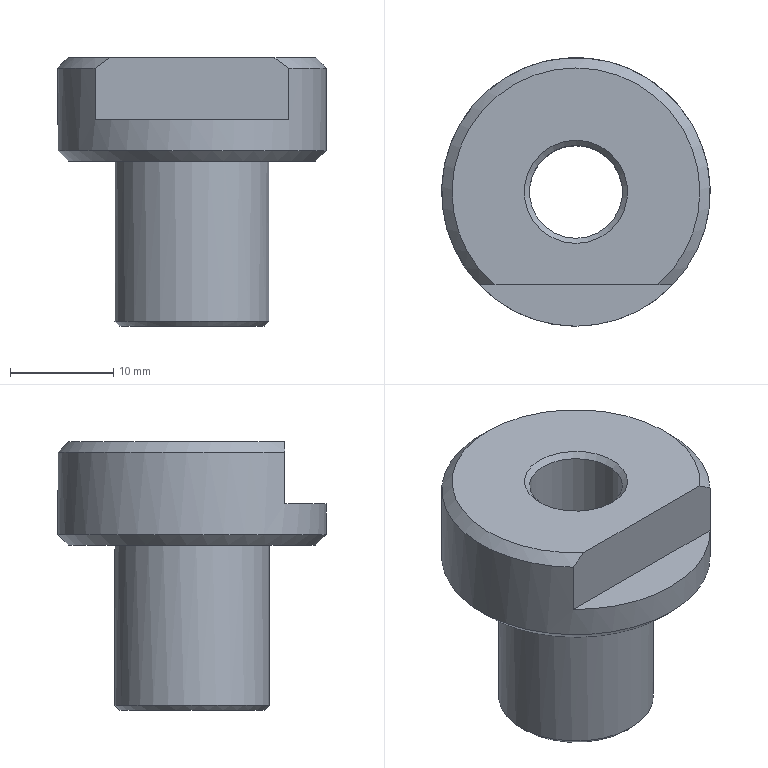Component | NX | DRILL_BUSHING | 1 solid | 13 faces | box 26 x 26 x 26 mm | volume 6089 mm3 | plane 5 | cone 5 | cylinder 3 | commonest cylinder face diameters 15 x1 26 x1 9 x1
STEP:
#1=CARTESIAN_POINT('',(0.,0.,0.));
#2=DIRECTION('',(0.,0.,1.));
#3=DIRECTION('',(1.,0.,0.));
#4=AXIS2_PLACEMENT_3D('',#1,#2,#3);
#5=CARTESIAN_POINT('',(376.101,-21.5,94.));
#6=VERTEX_POINT('',#5);
#7=CARTESIAN_POINT('',(376.101,-26.5,94.));
#8=DIRECTION('',(0.,0.,1.));
#9=DIRECTION('',(0.,1.,0.));
#10=AXIS2_PLACEMENT_3D('',#7,#8,#9);
#11=CIRCLE('',#10,5.);
#12=CARTESIAN_POINT('',(376.101,-26.5,94.));
#13=DIRECTION('',(0.,0.,-1.));
#14=DIRECTION('',(0.,1.,0.));
#15=AXIS2_PLACEMENT_3D('',#12,#13,#14);
#16=PLANE('',#15);
#17=CARTESIAN_POINT('',(5.,0.));
#18=CARTESIAN_POINT('',(5.,-8.66));
#19=CARTESIAN_POINT('',(-2.5,-4.33));
#20=CARTESIAN_POINT('',(-10.,-0.));
#21=CARTESIAN_POINT('',(-2.5,4.33));
#22=CARTESIAN_POINT('',(5.,8.66));
#23=CARTESIAN_POINT('',(5.,0.));
#24=(BOUNDED_CURVE()B_SPLINE_CURVE(2,(#17,#18,#19,#20,#21,#22,#23),.UNSPECIFIED.,.T.,.F.)B_SPLINE_CURVE_WITH_KNOTS((1,2,2,2,2,1),(-2.094,0.,2.094,4.189,6.283,8.378),.UNSPECIFIED.)CURVE()GEOMETRIC_REPRESENTATION_ITEM()RATIONAL_B_SPLINE_CURVE((1.,0.5,1.,0.5,1.,0.5,1.))REPRESENTATION_ITEM(''));
#25=(GEOMETRIC_REPRESENTATION_CONTEXT(2)PARAMETRIC_REPRESENTATION_CONTEXT()REPRESENTATION_CONTEXT('',''));
#26=DEFINITIONAL_REPRESENTATION('',(#24),#25);
#27=PCURVE('',#16,#26);
#28=CARTESIAN_POINT('',(376.101,-26.5,94.5));
#29=DIRECTION('',(0.,0.,-1.));
#30=DIRECTION('',(0.,1.,0.));
#31=AXIS2_PLACEMENT_3D('',#28,#29,#30);
#32=CONICAL_SURFACE('',#31,4.5,0.7854);
#33=CARTESIAN_POINT('',(6.283,0.5));
#34=DIRECTION('',(-1.,0.));
#35=VECTOR('',#34,1.);
#36=LINE('',#33,#35);
#37=(GEOMETRIC_REPRESENTATION_CONTEXT(2)PARAMETRIC_REPRESENTATION_CONTEXT()REPRESENTATION_CONTEXT('',''));
#38=DEFINITIONAL_REPRESENTATION('',(#36),#37);
#39=PCURVE('',#32,#38);
#40=SURFACE_CURVE('',#11,(#27,#39),.PCURVE_S1.);
#41=EDGE_CURVE('',#6,#6,#40,.T.);
#42=ORIENTED_EDGE('',*,*,#41,.T.);
#43=EDGE_LOOP('',(#42));
#44=FACE_BOUND('',#43,.T.);
#45=CARTESIAN_POINT('',(376.101,-19.5,94.));
#46=VERTEX_POINT('',#45);
#47=CARTESIAN_POINT('',(376.101,-26.5,94.));
#48=DIRECTION('',(0.,0.,-1.));
#49=DIRECTION('',(0.,1.,0.));
#50=AXIS2_PLACEMENT_3D('',#47,#48,#49);
#51=CIRCLE('',#50,7.);
#52=CARTESIAN_POINT('',(0.,0.));
#53=DIRECTION('',(1.,0.));
#54=AXIS2_PLACEMENT_2D('',#52,#53);
#55=CIRCLE('',#54,7.);
#56=(GEOMETRIC_REPRESENTATION_CONTEXT(2)PARAMETRIC_REPRESENTATION_CONTEXT()REPRESENTATION_CONTEXT('',''));
#57=DEFINITIONAL_REPRESENTATION('',(#55),#56);
#58=PCURVE('',#16,#57);
#59=CARTESIAN_POINT('',(376.101,-26.5,94.5));
#60=DIRECTION('',(0.,0.,1.));
#61=DIRECTION('',(0.,-1.,0.));
#62=AXIS2_PLACEMENT_3D('',#59,#60,#61);
#63=CONICAL_SURFACE('',#62,7.5,0.7854);
#64=CARTESIAN_POINT('',(9.425,-0.5));
#65=DIRECTION('',(-1.,0.));
#66=VECTOR('',#65,1.);
#67=LINE('',#64,#66);
#68=(GEOMETRIC_REPRESENTATION_CONTEXT(2)PARAMETRIC_REPRESENTATION_CONTEXT()REPRESENTATION_CONTEXT('',''));
#69=DEFINITIONAL_REPRESENTATION('',(#67),#68);
#70=PCURVE('',#63,#69);
#71=SURFACE_CURVE('',#51,(#58,#70),.PCURVE_S1.);
#72=EDGE_CURVE('',#46,#46,#71,.T.);
#73=ORIENTED_EDGE('',*,*,#72,.T.);
#74=EDGE_LOOP('',(#73));
#75=FACE_BOUND('',#74,.T.);
#76=ADVANCED_FACE('',(#44,#75),#16,.T.);
#77=CARTESIAN_POINT('',(376.101,-19.,94.5));
#78=VERTEX_POINT('',#77);
#79=CARTESIAN_POINT('',(376.101,-34.,94.5));
#80=VERTEX_POINT('',#79);
#81=CARTESIAN_POINT('',(376.101,-26.5,94.5));
#82=DIRECTION('',(0.,0.,1.));
#83=DIRECTION('',(0.,1.,0.));
#84=AXIS2_PLACEMENT_3D('',#81,#82,#83);
#85=CIRCLE('',#84,7.5);
#86=CARTESIAN_POINT('',(376.101,-26.5,94.));
#87=DIRECTION('',(0.,0.,1.));
#88=DIRECTION('',(0.,-1.,0.));
#89=AXIS2_PLACEMENT_3D('',#86,#87,#88);
#90=CYLINDRICAL_SURFACE('',#89,7.5);
#91=CARTESIAN_POINT('',(3.142,0.5));
#92=DIRECTION('',(1.,0.));
#93=VECTOR('',#92,1.);
#94=LINE('',#91,#93);
#95=(GEOMETRIC_REPRESENTATION_CONTEXT(2)PARAMETRIC_REPRESENTATION_CONTEXT()REPRESENTATION_CONTEXT('',''));
#96=DEFINITIONAL_REPRESENTATION('',(#94),#95);
#97=PCURVE('',#90,#96);
#98=CARTESIAN_POINT('',(3.142,0.));
#99=DIRECTION('',(1.,0.));
#100=VECTOR('',#99,1.);
#101=LINE('',#98,#100);
#102=(GEOMETRIC_REPRESENTATION_CONTEXT(2)PARAMETRIC_REPRESENTATION_CONTEXT()REPRESENTATION_CONTEXT('',''));
#103=DEFINITIONAL_REPRESENTATION('',(#101),#102);
#104=PCURVE('',#63,#103);
#105=SURFACE_CURVE('',#85,(#97,#104),.PCURVE_S1.);
#106=EDGE_CURVE('',#78,#80,#105,.T.);
#107=ORIENTED_EDGE('',*,*,#106,.T.);
#108=CARTESIAN_POINT('',(376.101,-34.,110.));
#109=VERTEX_POINT('',#108);
#110=CARTESIAN_POINT('',(376.101,-34.,94.5));
#111=CARTESIAN_POINT('',(376.101,-34.,110.));
#112=B_SPLINE_CURVE_WITH_KNOTS('',1,(#110,#111),.UNSPECIFIED.,.F.,.F.,(2,2),(0.5,16.),.PIECEWISE_BEZIER_KNOTS.);
#113=CARTESIAN_POINT('',(6.283,0.));
#114=DIRECTION('',(0.,1.));
#115=VECTOR('',#114,1.);
#116=LINE('',#113,#115);
#117=(GEOMETRIC_REPRESENTATION_CONTEXT(2)PARAMETRIC_REPRESENTATION_CONTEXT()REPRESENTATION_CONTEXT('',''));
#118=DEFINITIONAL_REPRESENTATION('',(#116),#117);
#119=PCURVE('',#90,#118);
#120=CARTESIAN_POINT('',(0.,0.));
#121=DIRECTION('',(0.,1.));
#122=VECTOR('',#121,1.);
#123=LINE('',#120,#122);
#124=(GEOMETRIC_REPRESENTATION_CONTEXT(2)PARAMETRIC_REPRESENTATION_CONTEXT()REPRESENTATION_CONTEXT('',''));
#125=DEFINITIONAL_REPRESENTATION('',(#123),#124);
#126=PCURVE('',#90,#125);
#127=SEAM_CURVE('',#112,(#119,#126),.PCURVE_S1.);
#128=EDGE_CURVE('',#80,#109,#127,.T.);
#129=ORIENTED_EDGE('',*,*,#128,.T.);
#130=CARTESIAN_POINT('',(376.101,-26.5,110.));
#131=DIRECTION('',(0.,0.,-1.));
#132=DIRECTION('',(0.,-1.,0.));
#133=AXIS2_PLACEMENT_3D('',#130,#131,#132);
#134=CIRCLE('',#133,7.5);
#135=CARTESIAN_POINT('',(6.283,16.));
#136=DIRECTION('',(-1.,0.));
#137=VECTOR('',#136,1.);
#138=LINE('',#135,#137);
#139=(GEOMETRIC_REPRESENTATION_CONTEXT(2)PARAMETRIC_REPRESENTATION_CONTEXT()REPRESENTATION_CONTEXT('',''));
#140=DEFINITIONAL_REPRESENTATION('',(#138),#139);
#141=PCURVE('',#90,#140);
#142=CARTESIAN_POINT('',(376.101,-26.5,110.));
#143=DIRECTION('',(0.,0.,-1.));
#144=DIRECTION('',(0.,1.,0.));
#145=AXIS2_PLACEMENT_3D('',#142,#143,#144);
#146=PLANE('',#145);
#147=CARTESIAN_POINT('',(0.,0.));
#148=DIRECTION('',(-1.,0.));
#149=AXIS2_PLACEMENT_2D('',#147,#148);
#150=CIRCLE('',#149,7.5);
#151=(GEOMETRIC_REPRESENTATION_CONTEXT(2)PARAMETRIC_REPRESENTATION_CONTEXT()REPRESENTATION_CONTEXT('',''));
#152=DEFINITIONAL_REPRESENTATION('',(#150),#151);
#153=PCURVE('',#146,#152);
#154=SURFACE_CURVE('',#134,(#141,#153),.PCURVE_S1.);
#155=EDGE_CURVE('',#109,#109,#154,.T.);
#156=ORIENTED_EDGE('',*,*,#155,.T.);
#157=ORIENTED_EDGE('',*,*,#128,.F.);
#158=CARTESIAN_POINT('',(376.101,-26.5,94.5));
#159=DIRECTION('',(0.,0.,1.));
#160=DIRECTION('',(0.,1.,0.));
#161=AXIS2_PLACEMENT_3D('',#158,#159,#160);
#162=CIRCLE('',#161,7.5);
#163=CARTESIAN_POINT('',(-3.142,0.5));
#164=DIRECTION('',(1.,0.));
#165=VECTOR('',#164,1.);
#166=LINE('',#163,#165);
#167=(GEOMETRIC_REPRESENTATION_CONTEXT(2)PARAMETRIC_REPRESENTATION_CONTEXT()REPRESENTATION_CONTEXT('',''));
#168=DEFINITIONAL_REPRESENTATION('',(#166),#167);
#169=PCURVE('',#90,#168);
#170=CARTESIAN_POINT('',(3.142,0.));
#171=DIRECTION('',(1.,0.));
#172=VECTOR('',#171,1.);
#173=LINE('',#170,#172);
#174=(GEOMETRIC_REPRESENTATION_CONTEXT(2)PARAMETRIC_REPRESENTATION_CONTEXT()REPRESENTATION_CONTEXT('',''));
#175=DEFINITIONAL_REPRESENTATION('',(#173),#174);
#176=PCURVE('',#63,#175);
#177=SURFACE_CURVE('',#162,(#169,#176),.PCURVE_S1.);
#178=EDGE_CURVE('',#80,#78,#177,.T.);
#179=ORIENTED_EDGE('',*,*,#178,.T.);
#180=EDGE_LOOP('',(#107,#129,#156,#157,#179));
#181=FACE_BOUND('',#180,.T.);
#182=ADVANCED_FACE('',(#181),#90,.T.);
#183=CARTESIAN_POINT('',(376.101,-31.5,120.));
#184=VERTEX_POINT('',#183);
#185=CARTESIAN_POINT('',(376.101,-26.5,120.));
#186=DIRECTION('',(0.,0.,-1.));
#187=DIRECTION('',(0.,-1.,0.));
#188=AXIS2_PLACEMENT_3D('',#185,#186,#187);
#189=CIRCLE('',#188,5.);
#190=CARTESIAN_POINT('',(376.101,-26.5,120.));
#191=DIRECTION('',(0.,0.,1.));
#192=DIRECTION('',(0.,-1.,0.));
#193=AXIS2_PLACEMENT_3D('',#190,#191,#192);
#194=PLANE('',#193);
#195=CARTESIAN_POINT('',(5.,0.));
#196=CARTESIAN_POINT('',(5.,-8.66));
#197=CARTESIAN_POINT('',(-2.5,-4.33));
#198=CARTESIAN_POINT('',(-10.,-0.));
#199=CARTESIAN_POINT('',(-2.5,4.33));
#200=CARTESIAN_POINT('',(5.,8.66));
#201=CARTESIAN_POINT('',(5.,0.));
#202=(BOUNDED_CURVE()B_SPLINE_CURVE(2,(#195,#196,#197,#198,#199,#200,#201),.UNSPECIFIED.,.T.,.F.)B_SPLINE_CURVE_WITH_KNOTS((1,2,2,2,2,1),(-2.094,0.,2.094,4.189,6.283,8.378),.UNSPECIFIED.)CURVE()GEOMETRIC_REPRESENTATION_ITEM()RATIONAL_B_SPLINE_CURVE((1.,0.5,1.,0.5,1.,0.5,1.))REPRESENTATION_ITEM(''));
#203=(GEOMETRIC_REPRESENTATION_CONTEXT(2)PARAMETRIC_REPRESENTATION_CONTEXT()REPRESENTATION_CONTEXT('',''));
#204=DEFINITIONAL_REPRESENTATION('',(#202),#203);
#205=PCURVE('',#194,#204);
#206=CARTESIAN_POINT('',(376.101,-26.5,120.));
#207=DIRECTION('',(0.,0.,1.));
#208=DIRECTION('',(0.,-1.,0.));
#209=AXIS2_PLACEMENT_3D('',#206,#207,#208);
#210=CONICAL_SURFACE('',#209,5.,0.7854);
#211=CARTESIAN_POINT('',(6.283,0.));
#212=DIRECTION('',(-1.,0.));
#213=VECTOR('',#212,1.);
#214=LINE('',#211,#213);
#215=(GEOMETRIC_REPRESENTATION_CONTEXT(2)PARAMETRIC_REPRESENTATION_CONTEXT()REPRESENTATION_CONTEXT('',''));
#216=DEFINITIONAL_REPRESENTATION('',(#214),#215);
#217=PCURVE('',#210,#216);
#218=SURFACE_CURVE('',#189,(#205,#217),.PCURVE_S1.);
#219=EDGE_CURVE('',#184,#184,#218,.T.);
#220=ORIENTED_EDGE('',*,*,#219,.T.);
#221=EDGE_LOOP('',(#220));
#222=FACE_BOUND('',#221,.T.);
#223=CARTESIAN_POINT('',(384.038,-35.5,120.));
#224=VERTEX_POINT('',#223);
#225=CARTESIAN_POINT('',(368.164,-35.5,120.));
#226=VERTEX_POINT('',#225);
#227=CARTESIAN_POINT('',(399.244,-35.5,120.));
#228=DIRECTION('',(-1.,0.,0.));
#229=VECTOR('',#228,1.);
#230=LINE('',#227,#229);
#231=CARTESIAN_POINT('',(9.,23.143));
#232=DIRECTION('',(0.,-1.));
#233=VECTOR('',#232,1.);
#234=LINE('',#231,#233);
#235=(GEOMETRIC_REPRESENTATION_CONTEXT(2)PARAMETRIC_REPRESENTATION_CONTEXT()REPRESENTATION_CONTEXT('',''));
#236=DEFINITIONAL_REPRESENTATION('',(#234),#235);
#237=PCURVE('',#194,#236);
#238=CARTESIAN_POINT('',(399.244,-35.5,114.));
#239=DIRECTION('',(0.,1.,0.));
#240=DIRECTION('',(0.,0.,1.));
#241=AXIS2_PLACEMENT_3D('',#238,#239,#240);
#242=PLANE('',#241);
#243=CARTESIAN_POINT('',(6.,0.));
#244=DIRECTION('',(0.,-1.));
#245=VECTOR('',#244,1.);
#246=LINE('',#243,#245);
#247=(GEOMETRIC_REPRESENTATION_CONTEXT(2)PARAMETRIC_REPRESENTATION_CONTEXT()REPRESENTATION_CONTEXT('',''));
#248=DEFINITIONAL_REPRESENTATION('',(#246),#247);
#249=PCURVE('',#242,#248);
#250=SURFACE_CURVE('',#230,(#237,#249),.PCURVE_S1.);
#251=EDGE_CURVE('',#224,#226,#250,.T.);
#252=ORIENTED_EDGE('',*,*,#251,.F.);
#253=CARTESIAN_POINT('',(376.101,-26.5,120.));
#254=DIRECTION('',(0.,0.,1.));
#255=DIRECTION('',(0.,-1.,0.));
#256=AXIS2_PLACEMENT_3D('',#253,#254,#255);
#257=CIRCLE('',#256,12.);
#258=CARTESIAN_POINT('',(0.,0.));
#259=DIRECTION('',(1.,0.));
#260=AXIS2_PLACEMENT_2D('',#258,#259);
#261=CIRCLE('',#260,12.);
#262=(GEOMETRIC_REPRESENTATION_CONTEXT(2)PARAMETRIC_REPRESENTATION_CONTEXT()REPRESENTATION_CONTEXT('',''));
#263=DEFINITIONAL_REPRESENTATION('',(#261),#262);
#264=PCURVE('',#194,#263);
#265=CARTESIAN_POINT('',(376.101,-26.5,119.));
#266=DIRECTION('',(0.,0.,-1.));
#267=DIRECTION('',(0.,1.,0.));
#268=AXIS2_PLACEMENT_3D('',#265,#266,#267);
#269=CONICAL_SURFACE('',#268,13.,0.7854);
#270=CARTESIAN_POINT('',(9.425,-1.));
#271=DIRECTION('',(-1.,0.));
#272=VECTOR('',#271,1.);
#273=LINE('',#270,#272);
#274=(GEOMETRIC_REPRESENTATION_CONTEXT(2)PARAMETRIC_REPRESENTATION_CONTEXT()REPRESENTATION_CONTEXT('',''));
#275=DEFINITIONAL_REPRESENTATION('',(#273),#274);
#276=PCURVE('',#269,#275);
#277=SURFACE_CURVE('',#257,(#264,#276),.PCURVE_S1.);
#278=EDGE_CURVE('',#224,#226,#277,.T.);
#279=ORIENTED_EDGE('',*,*,#278,.T.);
#280=EDGE_LOOP('',(#252,#279));
#281=FACE_BOUND('',#280,.T.);
#282=ADVANCED_FACE('',(#222,#281),#194,.T.);
#283=CARTESIAN_POINT('',(376.101,-14.5,110.));
#284=VERTEX_POINT('',#283);
#285=CARTESIAN_POINT('',(376.101,-26.5,110.));
#286=DIRECTION('',(0.,0.,-1.));
#287=DIRECTION('',(0.,1.,0.));
#288=AXIS2_PLACEMENT_3D('',#285,#286,#287);
#289=CIRCLE('',#288,12.);
#290=CARTESIAN_POINT('',(0.,0.));
#291=DIRECTION('',(1.,0.));
#292=AXIS2_PLACEMENT_2D('',#290,#291);
#293=CIRCLE('',#292,12.);
#294=(GEOMETRIC_REPRESENTATION_CONTEXT(2)PARAMETRIC_REPRESENTATION_CONTEXT()REPRESENTATION_CONTEXT('',''));
#295=DEFINITIONAL_REPRESENTATION('',(#293),#294);
#296=PCURVE('',#146,#295);
#297=CARTESIAN_POINT('',(376.101,-26.5,111.));
#298=DIRECTION('',(0.,0.,1.));
#299=DIRECTION('',(0.,-1.,0.));
#300=AXIS2_PLACEMENT_3D('',#297,#298,#299);
#301=CONICAL_SURFACE('',#300,13.,0.7854);
#302=CARTESIAN_POINT('',(9.425,-1.));
#303=DIRECTION('',(-1.,0.));
#304=VECTOR('',#303,1.);
#305=LINE('',#302,#304);
#306=(GEOMETRIC_REPRESENTATION_CONTEXT(2)PARAMETRIC_REPRESENTATION_CONTEXT()REPRESENTATION_CONTEXT('',''));
#307=DEFINITIONAL_REPRESENTATION('',(#305),#306);
#308=PCURVE('',#301,#307);
#309=SURFACE_CURVE('',#289,(#296,#308),.PCURVE_S1.);
#310=EDGE_CURVE('',#284,#284,#309,.T.);
#311=ORIENTED_EDGE('',*,*,#310,.T.);
#312=EDGE_LOOP('',(#311));
#313=FACE_BOUND('',#312,.T.);
#314=ORIENTED_EDGE('',*,*,#155,.F.);
#315=EDGE_LOOP('',(#314));
#316=FACE_BOUND('',#315,.T.);
#317=ADVANCED_FACE('',(#313,#316),#146,.T.);
#318=CARTESIAN_POINT('',(376.101,-13.5,111.));
#319=VERTEX_POINT('',#318);
#320=CARTESIAN_POINT('',(385.482,-35.5,111.));
#321=VERTEX_POINT('',#320);
#322=CARTESIAN_POINT('',(376.101,-26.5,111.));
#323=DIRECTION('',(0.,0.,1.));
#324=DIRECTION('',(0.,1.,0.));
#325=AXIS2_PLACEMENT_3D('',#322,#323,#324);
#326=CIRCLE('',#325,13.);
#327=CARTESIAN_POINT('',(376.101,-26.5,110.));
#328=DIRECTION('',(0.,0.,1.));
#329=DIRECTION('',(0.,-1.,0.));
#330=AXIS2_PLACEMENT_3D('',#327,#328,#329);
#331=CYLINDRICAL_SURFACE('',#330,13.);
#332=CARTESIAN_POINT('',(3.142,1.));
#333=DIRECTION('',(1.,0.));
#334=VECTOR('',#333,1.);
#335=LINE('',#332,#334);
#336=(GEOMETRIC_REPRESENTATION_CONTEXT(2)PARAMETRIC_REPRESENTATION_CONTEXT()REPRESENTATION_CONTEXT('',''));
#337=DEFINITIONAL_REPRESENTATION('',(#335),#336);
#338=PCURVE('',#331,#337);
#339=CARTESIAN_POINT('',(3.142,0.));
#340=DIRECTION('',(1.,-0.));
#341=VECTOR('',#340,1.);
#342=LINE('',#339,#341);
#343=(GEOMETRIC_REPRESENTATION_CONTEXT(2)PARAMETRIC_REPRESENTATION_CONTEXT()REPRESENTATION_CONTEXT('',''));
#344=DEFINITIONAL_REPRESENTATION('',(#342),#343);
#345=PCURVE('',#301,#344);
#346=SURFACE_CURVE('',#326,(#338,#345),.PCURVE_S1.);
#347=EDGE_CURVE('',#319,#321,#346,.T.);
#348=ORIENTED_EDGE('',*,*,#347,.T.);
#349=CARTESIAN_POINT('',(385.482,-35.5,114.));
#350=VERTEX_POINT('',#349);
#351=CARTESIAN_POINT('',(385.482,-35.5,111.));
#352=CARTESIAN_POINT('',(385.482,-35.5,114.));
#353=B_SPLINE_CURVE_WITH_KNOTS('',1,(#351,#352),.UNSPECIFIED.,.F.,.F.,(2,2),(1.,4.),.PIECEWISE_BEZIER_KNOTS.);
#354=CARTESIAN_POINT('',(7.089,0.));
#355=DIRECTION('',(0.,1.));
#356=VECTOR('',#355,1.);
#357=LINE('',#354,#356);
#358=(GEOMETRIC_REPRESENTATION_CONTEXT(2)PARAMETRIC_REPRESENTATION_CONTEXT()REPRESENTATION_CONTEXT('',''));
#359=DEFINITIONAL_REPRESENTATION('',(#357),#358);
#360=PCURVE('',#331,#359);
#361=CARTESIAN_POINT('',(0.8061,0.));
#362=DIRECTION('',(0.,1.));
#363=VECTOR('',#362,1.);
#364=LINE('',#361,#363);
#365=(GEOMETRIC_REPRESENTATION_CONTEXT(2)PARAMETRIC_REPRESENTATION_CONTEXT()REPRESENTATION_CONTEXT('',''));
#366=DEFINITIONAL_REPRESENTATION('',(#364),#365);
#367=PCURVE('',#331,#366);
#368=SEAM_CURVE('',#353,(#360,#367),.PCURVE_S1.);
#369=EDGE_CURVE('',#321,#350,#368,.T.);
#370=ORIENTED_EDGE('',*,*,#369,.T.);
#371=CARTESIAN_POINT('',(366.72,-35.5,114.));
#372=VERTEX_POINT('',#371);
#373=CARTESIAN_POINT('',(376.101,-26.5,114.));
#374=DIRECTION('',(0.,0.,-1.));
#375=DIRECTION('',(0.,-1.,0.));
#376=AXIS2_PLACEMENT_3D('',#373,#374,#375);
#377=CIRCLE('',#376,13.);
#378=CARTESIAN_POINT('',(12.566,4.));
#379=DIRECTION('',(-1.,0.));
#380=VECTOR('',#379,1.);
#381=LINE('',#378,#380);
#382=(GEOMETRIC_REPRESENTATION_CONTEXT(2)PARAMETRIC_REPRESENTATION_CONTEXT()REPRESENTATION_CONTEXT('',''));
#383=DEFINITIONAL_REPRESENTATION('',(#381),#382);
#384=PCURVE('',#331,#383);
#385=CARTESIAN_POINT('',(376.101,-26.5,114.));
#386=DIRECTION('',(0.,0.,1.));
#387=DIRECTION('',(0.,-1.,0.));
#388=AXIS2_PLACEMENT_3D('',#385,#386,#387);
#389=PLANE('',#388);
#390=CARTESIAN_POINT('',(13.,0.));
#391=CARTESIAN_POINT('',(13.,-22.517));
#392=CARTESIAN_POINT('',(-6.5,-11.258));
#393=CARTESIAN_POINT('',(-26.,-0.));
#394=CARTESIAN_POINT('',(-6.5,11.258));
#395=CARTESIAN_POINT('',(13.,22.517));
#396=CARTESIAN_POINT('',(13.,0.));
#397=(BOUNDED_CURVE()B_SPLINE_CURVE(2,(#390,#391,#392,#393,#394,#395,#396),.UNSPECIFIED.,.T.,.F.)B_SPLINE_CURVE_WITH_KNOTS((1,2,2,2,2,1),(-2.094,0.,2.094,4.189,6.283,8.378),.UNSPECIFIED.)CURVE()GEOMETRIC_REPRESENTATION_ITEM()RATIONAL_B_SPLINE_CURVE((1.,0.5,1.,0.5,1.,0.5,1.))REPRESENTATION_ITEM(''));
#398=(GEOMETRIC_REPRESENTATION_CONTEXT(2)PARAMETRIC_REPRESENTATION_CONTEXT()REPRESENTATION_CONTEXT('',''));
#399=DEFINITIONAL_REPRESENTATION('',(#397),#398);
#400=PCURVE('',#389,#399);
#401=SURFACE_CURVE('',#377,(#384,#400),.PCURVE_S1.);
#402=EDGE_CURVE('',#350,#372,#401,.T.);
#403=ORIENTED_EDGE('',*,*,#402,.T.);
#404=CARTESIAN_POINT('',(366.72,-35.5,119.));
#405=VERTEX_POINT('',#404);
#406=CARTESIAN_POINT('',(366.72,-35.5,110.));
#407=DIRECTION('',(0.,0.,-1.));
#408=VECTOR('',#407,1.);
#409=LINE('',#406,#408);
#410=CARTESIAN_POINT('',(5.477,0.));
#411=DIRECTION('',(0.,-1.));
#412=VECTOR('',#411,1.);
#413=LINE('',#410,#412);
#414=(GEOMETRIC_REPRESENTATION_CONTEXT(2)PARAMETRIC_REPRESENTATION_CONTEXT()REPRESENTATION_CONTEXT('',''));
#415=DEFINITIONAL_REPRESENTATION('',(#413),#414);
#416=PCURVE('',#331,#415);
#417=CARTESIAN_POINT('',(-4.,-32.524));
#418=DIRECTION('',(-1.,0.));
#419=VECTOR('',#418,1.);
#420=LINE('',#417,#419);
#421=(GEOMETRIC_REPRESENTATION_CONTEXT(2)PARAMETRIC_REPRESENTATION_CONTEXT()REPRESENTATION_CONTEXT('',''));
#422=DEFINITIONAL_REPRESENTATION('',(#420),#421);
#423=PCURVE('',#242,#422);
#424=SURFACE_CURVE('',#409,(#416,#423),.PCURVE_S1.);
#425=EDGE_CURVE('',#405,#372,#424,.T.);
#426=ORIENTED_EDGE('',*,*,#425,.F.);
#427=CARTESIAN_POINT('',(385.482,-35.5,119.));
#428=VERTEX_POINT('',#427);
#429=CARTESIAN_POINT('',(376.101,-26.5,119.));
#430=DIRECTION('',(0.,0.,-1.));
#431=DIRECTION('',(0.,-1.,0.));
#432=AXIS2_PLACEMENT_3D('',#429,#430,#431);
#433=CIRCLE('',#432,13.);
#434=CARTESIAN_POINT('',(6.283,9.));
#435=DIRECTION('',(-1.,0.));
#436=VECTOR('',#435,1.);
#437=LINE('',#434,#436);
#438=(GEOMETRIC_REPRESENTATION_CONTEXT(2)PARAMETRIC_REPRESENTATION_CONTEXT()REPRESENTATION_CONTEXT('',''));
#439=DEFINITIONAL_REPRESENTATION('',(#437),#438);
#440=PCURVE('',#331,#439);
#441=CARTESIAN_POINT('',(3.142,0.));
#442=DIRECTION('',(1.,0.));
#443=VECTOR('',#442,1.);
#444=LINE('',#441,#443);
#445=(GEOMETRIC_REPRESENTATION_CONTEXT(2)PARAMETRIC_REPRESENTATION_CONTEXT()REPRESENTATION_CONTEXT('',''));
#446=DEFINITIONAL_REPRESENTATION('',(#444),#445);
#447=PCURVE('',#269,#446);
#448=SURFACE_CURVE('',#433,(#440,#447),.PCURVE_S1.);
#449=EDGE_CURVE('',#405,#428,#448,.T.);
#450=ORIENTED_EDGE('',*,*,#449,.T.);
#451=CARTESIAN_POINT('',(385.482,-35.5,110.));
#452=DIRECTION('',(0.,0.,1.));
#453=VECTOR('',#452,1.);
#454=LINE('',#451,#453);
#455=CARTESIAN_POINT('',(0.8061,0.));
#456=DIRECTION('',(0.,1.));
#457=VECTOR('',#456,1.);
#458=LINE('',#455,#457);
#459=(GEOMETRIC_REPRESENTATION_CONTEXT(2)PARAMETRIC_REPRESENTATION_CONTEXT()REPRESENTATION_CONTEXT('',''));
#460=DEFINITIONAL_REPRESENTATION('',(#458),#459);
#461=PCURVE('',#331,#460);
#462=CARTESIAN_POINT('',(-4.,-13.762));
#463=DIRECTION('',(1.,0.));
#464=VECTOR('',#463,1.);
#465=LINE('',#462,#464);
#466=(GEOMETRIC_REPRESENTATION_CONTEXT(2)PARAMETRIC_REPRESENTATION_CONTEXT()REPRESENTATION_CONTEXT('',''));
#467=DEFINITIONAL_REPRESENTATION('',(#465),#466);
#468=PCURVE('',#242,#467);
#469=SURFACE_CURVE('',#454,(#461,#468),.PCURVE_S1.);
#470=EDGE_CURVE('',#350,#428,#469,.T.);
#471=ORIENTED_EDGE('',*,*,#470,.F.);
#472=ORIENTED_EDGE('',*,*,#369,.F.);
#473=CARTESIAN_POINT('',(376.101,-26.5,111.));
#474=DIRECTION('',(0.,0.,1.));
#475=DIRECTION('',(0.,1.,0.));
#476=AXIS2_PLACEMENT_3D('',#473,#474,#475);
#477=CIRCLE('',#476,13.);
#478=CARTESIAN_POINT('',(-3.142,1.));
#479=DIRECTION('',(1.,0.));
#480=VECTOR('',#479,1.);
#481=LINE('',#478,#480);
#482=(GEOMETRIC_REPRESENTATION_CONTEXT(2)PARAMETRIC_REPRESENTATION_CONTEXT()REPRESENTATION_CONTEXT('',''));
#483=DEFINITIONAL_REPRESENTATION('',(#481),#482);
#484=PCURVE('',#331,#483);
#485=CARTESIAN_POINT('',(3.142,-0.));
#486=DIRECTION('',(1.,0.));
#487=VECTOR('',#486,1.);
#488=LINE('',#485,#487);
#489=(GEOMETRIC_REPRESENTATION_CONTEXT(2)PARAMETRIC_REPRESENTATION_CONTEXT()REPRESENTATION_CONTEXT('',''));
#490=DEFINITIONAL_REPRESENTATION('',(#488),#489);
#491=PCURVE('',#301,#490);
#492=SURFACE_CURVE('',#477,(#484,#491),.PCURVE_S1.);
#493=EDGE_CURVE('',#321,#319,#492,.T.);
#494=ORIENTED_EDGE('',*,*,#493,.T.);
#495=EDGE_LOOP('',(#348,#370,#403,#426,#450,#471,#472,#494));
#496=FACE_BOUND('',#495,.T.);
#497=ADVANCED_FACE('',(#496),#331,.T.);
#498=CARTESIAN_POINT('',(376.101,-22.,119.5));
#499=VERTEX_POINT('',#498);
#500=CARTESIAN_POINT('',(376.101,-31.,119.5));
#501=VERTEX_POINT('',#500);
#502=CARTESIAN_POINT('',(376.101,-26.5,119.5));
#503=DIRECTION('',(0.,0.,1.));
#504=DIRECTION('',(0.,-1.,0.));
#505=AXIS2_PLACEMENT_3D('',#502,#503,#504);
#506=CIRCLE('',#505,4.5);
#507=CARTESIAN_POINT('',(376.101,-26.5,120.));
#508=DIRECTION('',(0.,0.,-1.));
#509=DIRECTION('',(0.,1.,0.));
#510=AXIS2_PLACEMENT_3D('',#507,#508,#509);
#511=CYLINDRICAL_SURFACE('',#510,4.5);
#512=CARTESIAN_POINT('',(9.425,0.5));
#513=DIRECTION('',(-1.,0.));
#514=VECTOR('',#513,1.);
#515=LINE('',#512,#514);
#516=(GEOMETRIC_REPRESENTATION_CONTEXT(2)PARAMETRIC_REPRESENTATION_CONTEXT()REPRESENTATION_CONTEXT('',''));
#517=DEFINITIONAL_REPRESENTATION('',(#515),#516);
#518=PCURVE('',#511,#517);
#519=CARTESIAN_POINT('',(0.,-0.5));
#520=DIRECTION('',(1.,0.));
#521=VECTOR('',#520,1.);
#522=LINE('',#519,#521);
#523=(GEOMETRIC_REPRESENTATION_CONTEXT(2)PARAMETRIC_REPRESENTATION_CONTEXT()REPRESENTATION_CONTEXT('',''));
#524=DEFINITIONAL_REPRESENTATION('',(#522),#523);
#525=PCURVE('',#210,#524);
#526=SURFACE_CURVE('',#506,(#518,#525),.PCURVE_S1.);
#527=EDGE_CURVE('',#499,#501,#526,.T.);
#528=ORIENTED_EDGE('',*,*,#527,.F.);
#529=CARTESIAN_POINT('',(376.101,-22.,94.5));
#530=VERTEX_POINT('',#529);
#531=CARTESIAN_POINT('',(376.101,-22.,119.5));
#532=CARTESIAN_POINT('',(376.101,-22.,94.5));
#533=B_SPLINE_CURVE_WITH_KNOTS('',1,(#531,#532),.UNSPECIFIED.,.F.,.F.,(2,2),(0.5,25.5),.PIECEWISE_BEZIER_KNOTS.);
#534=CARTESIAN_POINT('',(6.283,0.));
#535=DIRECTION('',(0.,1.));
#536=VECTOR('',#535,1.);
#537=LINE('',#534,#536);
#538=(GEOMETRIC_REPRESENTATION_CONTEXT(2)PARAMETRIC_REPRESENTATION_CONTEXT()REPRESENTATION_CONTEXT('',''));
#539=DEFINITIONAL_REPRESENTATION('',(#537),#538);
#540=PCURVE('',#511,#539);
#541=CARTESIAN_POINT('',(0.,0.));
#542=DIRECTION('',(0.,1.));
#543=VECTOR('',#542,1.);
#544=LINE('',#541,#543);
#545=(GEOMETRIC_REPRESENTATION_CONTEXT(2)PARAMETRIC_REPRESENTATION_CONTEXT()REPRESENTATION_CONTEXT('',''));
#546=DEFINITIONAL_REPRESENTATION('',(#544),#545);
#547=PCURVE('',#511,#546);
#548=SEAM_CURVE('',#533,(#540,#547),.PCURVE_S1.);
#549=EDGE_CURVE('',#499,#530,#548,.T.);
#550=ORIENTED_EDGE('',*,*,#549,.T.);
#551=CARTESIAN_POINT('',(376.101,-26.5,94.5));
#552=DIRECTION('',(0.,0.,-1.));
#553=DIRECTION('',(0.,1.,0.));
#554=AXIS2_PLACEMENT_3D('',#551,#552,#553);
#555=CIRCLE('',#554,4.5);
#556=CARTESIAN_POINT('',(0.,25.5));
#557=DIRECTION('',(1.,0.));
#558=VECTOR('',#557,1.);
#559=LINE('',#556,#558);
#560=(GEOMETRIC_REPRESENTATION_CONTEXT(2)PARAMETRIC_REPRESENTATION_CONTEXT()REPRESENTATION_CONTEXT('',''));
#561=DEFINITIONAL_REPRESENTATION('',(#559),#560);
#562=PCURVE('',#511,#561);
#563=CARTESIAN_POINT('',(0.,0.));
#564=DIRECTION('',(1.,0.));
#565=VECTOR('',#564,1.);
#566=LINE('',#563,#565);
#567=(GEOMETRIC_REPRESENTATION_CONTEXT(2)PARAMETRIC_REPRESENTATION_CONTEXT()REPRESENTATION_CONTEXT('',''));
#568=DEFINITIONAL_REPRESENTATION('',(#566),#567);
#569=PCURVE('',#32,#568);
#570=SURFACE_CURVE('',#555,(#562,#569),.PCURVE_S1.);
#571=EDGE_CURVE('',#530,#530,#570,.T.);
#572=ORIENTED_EDGE('',*,*,#571,.F.);
#573=ORIENTED_EDGE('',*,*,#549,.F.);
#574=CARTESIAN_POINT('',(376.101,-26.5,119.5));
#575=DIRECTION('',(0.,0.,1.));
#576=DIRECTION('',(0.,-1.,0.));
#577=AXIS2_PLACEMENT_3D('',#574,#575,#576);
#578=CIRCLE('',#577,4.5);
#579=CARTESIAN_POINT('',(3.142,0.5));
#580=DIRECTION('',(-1.,0.));
#581=VECTOR('',#580,1.);
#582=LINE('',#579,#581);
#583=(GEOMETRIC_REPRESENTATION_CONTEXT(2)PARAMETRIC_REPRESENTATION_CONTEXT()REPRESENTATION_CONTEXT('',''));
#584=DEFINITIONAL_REPRESENTATION('',(#582),#583);
#585=PCURVE('',#511,#584);
#586=CARTESIAN_POINT('',(0.,-0.5));
#587=DIRECTION('',(1.,0.));
#588=VECTOR('',#587,1.);
#589=LINE('',#586,#588);
#590=(GEOMETRIC_REPRESENTATION_CONTEXT(2)PARAMETRIC_REPRESENTATION_CONTEXT()REPRESENTATION_CONTEXT('',''));
#591=DEFINITIONAL_REPRESENTATION('',(#589),#590);
#592=PCURVE('',#210,#591);
#593=SURFACE_CURVE('',#578,(#585,#592),.PCURVE_S1.);
#594=EDGE_CURVE('',#501,#499,#593,.T.);
#595=ORIENTED_EDGE('',*,*,#594,.F.);
#596=EDGE_LOOP('',(#528,#550,#572,#573,#595));
#597=FACE_BOUND('',#596,.F.);
#598=ADVANCED_FACE('',(#597),#511,.F.);
#599=ORIENTED_EDGE('',*,*,#470,.T.);
#600=CARTESIAN_POINT('',(385.482,-35.5,119.));
#601=CARTESIAN_POINT('',(385.007,-35.5,119.343));
#602=CARTESIAN_POINT('',(384.527,-35.5,119.677));
#603=CARTESIAN_POINT('',(384.038,-35.5,120.));
#604=B_SPLINE_CURVE_WITH_KNOTS('',3,(#600,#601,#602,#603),.UNSPECIFIED.,.F.,.F.,(4,4),(0.,1.),.PIECEWISE_BEZIER_KNOTS.);
#605=CARTESIAN_POINT('',(5.,-13.762));
#606=CARTESIAN_POINT('',(5.343,-14.237));
#607=CARTESIAN_POINT('',(5.677,-14.717));
#608=CARTESIAN_POINT('',(6.,-15.206));
#609=B_SPLINE_CURVE_WITH_KNOTS('',3,(#605,#606,#607,#608),.UNSPECIFIED.,.F.,.F.,(4,4),(0.,1.),.PIECEWISE_BEZIER_KNOTS.);
#610=(GEOMETRIC_REPRESENTATION_CONTEXT(2)PARAMETRIC_REPRESENTATION_CONTEXT()REPRESENTATION_CONTEXT('',''));
#611=DEFINITIONAL_REPRESENTATION('',(#609),#610);
#612=PCURVE('',#242,#611);
#613=CARTESIAN_POINT('',(8.619,0.));
#614=CARTESIAN_POINT('',(8.702,-1.));
#615=B_SPLINE_CURVE_WITH_KNOTS('',1,(#613,#614),.UNSPECIFIED.,.F.,.F.,(2,2),(0.,1.),.PIECEWISE_BEZIER_KNOTS.);
#616=(GEOMETRIC_REPRESENTATION_CONTEXT(2)PARAMETRIC_REPRESENTATION_CONTEXT()REPRESENTATION_CONTEXT('',''));
#617=DEFINITIONAL_REPRESENTATION('',(#615),#616);
#618=PCURVE('',#269,#617);
#619=SURFACE_CURVE('',#604,(#612,#618),.PCURVE_S1.);
#620=EDGE_CURVE('',#428,#224,#619,.T.);
#621=ORIENTED_EDGE('',*,*,#620,.T.);
#622=ORIENTED_EDGE('',*,*,#251,.T.);
#623=CARTESIAN_POINT('',(368.164,-35.5,120.));
#624=CARTESIAN_POINT('',(367.676,-35.5,119.677));
#625=CARTESIAN_POINT('',(367.195,-35.5,119.343));
#626=CARTESIAN_POINT('',(366.72,-35.5,119.));
#627=B_SPLINE_CURVE_WITH_KNOTS('',3,(#623,#624,#625,#626),.UNSPECIFIED.,.F.,.F.,(4,4),(0.,1.),.PIECEWISE_BEZIER_KNOTS.);
#628=CARTESIAN_POINT('',(6.,-31.08));
#629=CARTESIAN_POINT('',(5.677,-31.568));
#630=CARTESIAN_POINT('',(5.343,-32.049));
#631=CARTESIAN_POINT('',(5.,-32.524));
#632=B_SPLINE_CURVE_WITH_KNOTS('',3,(#628,#629,#630,#631),.UNSPECIFIED.,.F.,.F.,(4,4),(0.,1.),.PIECEWISE_BEZIER_KNOTS.);
#633=(GEOMETRIC_REPRESENTATION_CONTEXT(2)PARAMETRIC_REPRESENTATION_CONTEXT()REPRESENTATION_CONTEXT('',''));
#634=DEFINITIONAL_REPRESENTATION('',(#632),#633);
#635=PCURVE('',#242,#634);
#636=CARTESIAN_POINT('',(3.864,-1.));
#637=CARTESIAN_POINT('',(3.948,0.));
#638=B_SPLINE_CURVE_WITH_KNOTS('',1,(#636,#637),.UNSPECIFIED.,.F.,.F.,(2,2),(0.,1.),.PIECEWISE_BEZIER_KNOTS.);
#639=(GEOMETRIC_REPRESENTATION_CONTEXT(2)PARAMETRIC_REPRESENTATION_CONTEXT()REPRESENTATION_CONTEXT('',''));
#640=DEFINITIONAL_REPRESENTATION('',(#638),#639);
#641=PCURVE('',#269,#640);
#642=SURFACE_CURVE('',#627,(#635,#641),.PCURVE_S1.);
#643=EDGE_CURVE('',#226,#405,#642,.T.);
#644=ORIENTED_EDGE('',*,*,#643,.T.);
#645=ORIENTED_EDGE('',*,*,#425,.T.);
#646=CARTESIAN_POINT('',(399.244,-35.5,114.));
#647=DIRECTION('',(1.,0.,0.));
#648=VECTOR('',#647,1.);
#649=LINE('',#646,#648);
#650=CARTESIAN_POINT('',(0.,0.));
#651=DIRECTION('',(0.,1.));
#652=VECTOR('',#651,1.);
#653=LINE('',#650,#652);
#654=(GEOMETRIC_REPRESENTATION_CONTEXT(2)PARAMETRIC_REPRESENTATION_CONTEXT()REPRESENTATION_CONTEXT('',''));
#655=DEFINITIONAL_REPRESENTATION('',(#653),#654);
#656=PCURVE('',#242,#655);
#657=CARTESIAN_POINT('',(9.,23.143));
#658=DIRECTION('',(0.,1.));
#659=VECTOR('',#658,1.);
#660=LINE('',#657,#659);
#661=(GEOMETRIC_REPRESENTATION_CONTEXT(2)PARAMETRIC_REPRESENTATION_CONTEXT()REPRESENTATION_CONTEXT('',''));
#662=DEFINITIONAL_REPRESENTATION('',(#660),#661);
#663=PCURVE('',#389,#662);
#664=SURFACE_CURVE('',#649,(#656,#663),.PCURVE_S1.);
#665=EDGE_CURVE('',#372,#350,#664,.T.);
#666=ORIENTED_EDGE('',*,*,#665,.T.);
#667=EDGE_LOOP('',(#599,#621,#622,#644,#645,#666));
#668=FACE_BOUND('',#667,.T.);
#669=ADVANCED_FACE('',(#668),#242,.F.);
#670=ORIENTED_EDGE('',*,*,#665,.F.);
#671=ORIENTED_EDGE('',*,*,#402,.F.);
#672=EDGE_LOOP('',(#670,#671));
#673=FACE_BOUND('',#672,.T.);
#674=ADVANCED_FACE('',(#673),#389,.T.);
#675=ORIENTED_EDGE('',*,*,#310,.F.);
#676=CARTESIAN_POINT('',(376.101,-14.5,110.));
#677=CARTESIAN_POINT('',(376.101,-13.5,111.));
#678=B_SPLINE_CURVE_WITH_KNOTS('',1,(#676,#677),.UNSPECIFIED.,.F.,.F.,(2,2),(-1.414,0.),.PIECEWISE_BEZIER_KNOTS.);
#679=CARTESIAN_POINT('',(9.425,0.));
#680=DIRECTION('',(0.,1.));
#681=VECTOR('',#680,1.);
#682=LINE('',#679,#681);
#683=(GEOMETRIC_REPRESENTATION_CONTEXT(2)PARAMETRIC_REPRESENTATION_CONTEXT()REPRESENTATION_CONTEXT('',''));
#684=DEFINITIONAL_REPRESENTATION('',(#682),#683);
#685=PCURVE('',#301,#684);
#686=CARTESIAN_POINT('',(3.142,0.));
#687=DIRECTION('',(0.,1.));
#688=VECTOR('',#687,1.);
#689=LINE('',#686,#688);
#690=(GEOMETRIC_REPRESENTATION_CONTEXT(2)PARAMETRIC_REPRESENTATION_CONTEXT()REPRESENTATION_CONTEXT('',''));
#691=DEFINITIONAL_REPRESENTATION('',(#689),#690);
#692=PCURVE('',#301,#691);
#693=SEAM_CURVE('',#678,(#685,#692),.PCURVE_S1.);
#694=EDGE_CURVE('',#284,#319,#693,.T.);
#695=ORIENTED_EDGE('',*,*,#694,.T.);
#696=ORIENTED_EDGE('',*,*,#493,.F.);
#697=ORIENTED_EDGE('',*,*,#347,.F.);
#698=ORIENTED_EDGE('',*,*,#694,.F.);
#699=EDGE_LOOP('',(#675,#695,#696,#697,#698));
#700=FACE_BOUND('',#699,.T.);
#701=ADVANCED_FACE('',(#700),#301,.T.);
#702=ORIENTED_EDGE('',*,*,#643,.F.);
#703=ORIENTED_EDGE('',*,*,#278,.F.);
#704=ORIENTED_EDGE('',*,*,#620,.F.);
#705=ORIENTED_EDGE('',*,*,#449,.F.);
#706=EDGE_LOOP('',(#702,#703,#704,#705));
#707=FACE_BOUND('',#706,.T.);
#708=ADVANCED_FACE('',(#707),#269,.T.);
#709=ORIENTED_EDGE('',*,*,#527,.T.);
#710=CARTESIAN_POINT('',(376.101,-31.,119.5));
#711=CARTESIAN_POINT('',(376.101,-31.5,120.));
#712=B_SPLINE_CURVE_WITH_KNOTS('',1,(#710,#711),.UNSPECIFIED.,.F.,.F.,(2,2),(-0.7071,0.),.PIECEWISE_BEZIER_KNOTS.);
#713=CARTESIAN_POINT('',(6.283,0.));
#714=DIRECTION('',(0.,1.));
#715=VECTOR('',#714,1.);
#716=LINE('',#713,#715);
#717=(GEOMETRIC_REPRESENTATION_CONTEXT(2)PARAMETRIC_REPRESENTATION_CONTEXT()REPRESENTATION_CONTEXT('',''));
#718=DEFINITIONAL_REPRESENTATION('',(#716),#717);
#719=PCURVE('',#210,#718);
#720=CARTESIAN_POINT('',(0.,0.));
#721=DIRECTION('',(0.,1.));
#722=VECTOR('',#721,1.);
#723=LINE('',#720,#722);
#724=(GEOMETRIC_REPRESENTATION_CONTEXT(2)PARAMETRIC_REPRESENTATION_CONTEXT()REPRESENTATION_CONTEXT('',''));
#725=DEFINITIONAL_REPRESENTATION('',(#723),#724);
#726=PCURVE('',#210,#725);
#727=SEAM_CURVE('',#712,(#719,#726),.PCURVE_S1.);
#728=EDGE_CURVE('',#501,#184,#727,.T.);
#729=ORIENTED_EDGE('',*,*,#728,.T.);
#730=ORIENTED_EDGE('',*,*,#219,.T.);
#731=ORIENTED_EDGE('',*,*,#728,.F.);
#732=ORIENTED_EDGE('',*,*,#594,.T.);
#733=EDGE_LOOP('',(#709,#729,#730,#731,#732));
#734=FACE_BOUND('',#733,.F.);
#735=ADVANCED_FACE('',(#734),#210,.F.);
#736=ORIENTED_EDGE('',*,*,#41,.T.);
#737=CARTESIAN_POINT('',(376.101,-22.,94.5));
#738=CARTESIAN_POINT('',(376.101,-21.5,94.));
#739=B_SPLINE_CURVE_WITH_KNOTS('',1,(#737,#738),.UNSPECIFIED.,.F.,.F.,(2,2),(0.,0.7071),.PIECEWISE_BEZIER_KNOTS.);
#740=CARTESIAN_POINT('',(0.,0.));
#741=DIRECTION('',(0.,1.));
#742=VECTOR('',#741,1.);
#743=LINE('',#740,#742);
#744=(GEOMETRIC_REPRESENTATION_CONTEXT(2)PARAMETRIC_REPRESENTATION_CONTEXT()REPRESENTATION_CONTEXT('',''));
#745=DEFINITIONAL_REPRESENTATION('',(#743),#744);
#746=PCURVE('',#32,#745);
#747=CARTESIAN_POINT('',(6.283,0.));
#748=DIRECTION('',(0.,1.));
#749=VECTOR('',#748,1.);
#750=LINE('',#747,#749);
#751=(GEOMETRIC_REPRESENTATION_CONTEXT(2)PARAMETRIC_REPRESENTATION_CONTEXT()REPRESENTATION_CONTEXT('',''));
#752=DEFINITIONAL_REPRESENTATION('',(#750),#751);
#753=PCURVE('',#32,#752);
#754=SEAM_CURVE('',#739,(#746,#753),.PCURVE_S1.);
#755=EDGE_CURVE('',#530,#6,#754,.T.);
#756=ORIENTED_EDGE('',*,*,#755,.F.);
#757=ORIENTED_EDGE('',*,*,#571,.T.);
#758=ORIENTED_EDGE('',*,*,#755,.T.);
#759=EDGE_LOOP('',(#736,#756,#757,#758));
#760=FACE_BOUND('',#759,.F.);
#761=ADVANCED_FACE('',(#760),#32,.F.);
#762=ORIENTED_EDGE('',*,*,#72,.F.);
#763=CARTESIAN_POINT('',(376.101,-19.5,94.));
#764=CARTESIAN_POINT('',(376.101,-19.,94.5));
#765=B_SPLINE_CURVE_WITH_KNOTS('',1,(#763,#764),.UNSPECIFIED.,.F.,.F.,(2,2),(-0.7071,0.),.PIECEWISE_BEZIER_KNOTS.);
#766=CARTESIAN_POINT('',(9.425,0.));
#767=DIRECTION('',(0.,1.));
#768=VECTOR('',#767,1.);
#769=LINE('',#766,#768);
#770=(GEOMETRIC_REPRESENTATION_CONTEXT(2)PARAMETRIC_REPRESENTATION_CONTEXT()REPRESENTATION_CONTEXT('',''));
#771=DEFINITIONAL_REPRESENTATION('',(#769),#770);
#772=PCURVE('',#63,#771);
#773=CARTESIAN_POINT('',(3.142,0.));
#774=DIRECTION('',(0.,1.));
#775=VECTOR('',#774,1.);
#776=LINE('',#773,#775);
#777=(GEOMETRIC_REPRESENTATION_CONTEXT(2)PARAMETRIC_REPRESENTATION_CONTEXT()REPRESENTATION_CONTEXT('',''));
#778=DEFINITIONAL_REPRESENTATION('',(#776),#777);
#779=PCURVE('',#63,#778);
#780=SEAM_CURVE('',#765,(#772,#779),.PCURVE_S1.);
#781=EDGE_CURVE('',#46,#78,#780,.T.);
#782=ORIENTED_EDGE('',*,*,#781,.T.);
#783=ORIENTED_EDGE('',*,*,#178,.F.);
#784=ORIENTED_EDGE('',*,*,#106,.F.);
#785=ORIENTED_EDGE('',*,*,#781,.F.);
#786=EDGE_LOOP('',(#762,#782,#783,#784,#785));
#787=FACE_BOUND('',#786,.T.);
#788=ADVANCED_FACE('',(#787),#63,.T.);
#789=CLOSED_SHELL('',(#76,#182,#282,#317,#497,#598,#669,#674,#701,#708,#735,#761,#788));
#790=MANIFOLD_SOLID_BREP('',#789);
#791=(LENGTH_UNIT()NAMED_UNIT(*)SI_UNIT(.MILLI.,.METRE.));
#792=UNCERTAINTY_MEASURE_WITH_UNIT(LENGTH_MEASURE(0.005),#791,'','');
#793=(NAMED_UNIT(*)PLANE_ANGLE_UNIT()SI_UNIT($,.RADIAN.));
#794=(NAMED_UNIT(*)SI_UNIT($,.STERADIAN.)SOLID_ANGLE_UNIT());
#795=(GEOMETRIC_REPRESENTATION_CONTEXT(3)GLOBAL_UNCERTAINTY_ASSIGNED_CONTEXT((#792))GLOBAL_UNIT_ASSIGNED_CONTEXT((#791,#793,#794))REPRESENTATION_CONTEXT('',''));
#796=ADVANCED_BREP_SHAPE_REPRESENTATION('',(#4,#790),#795);